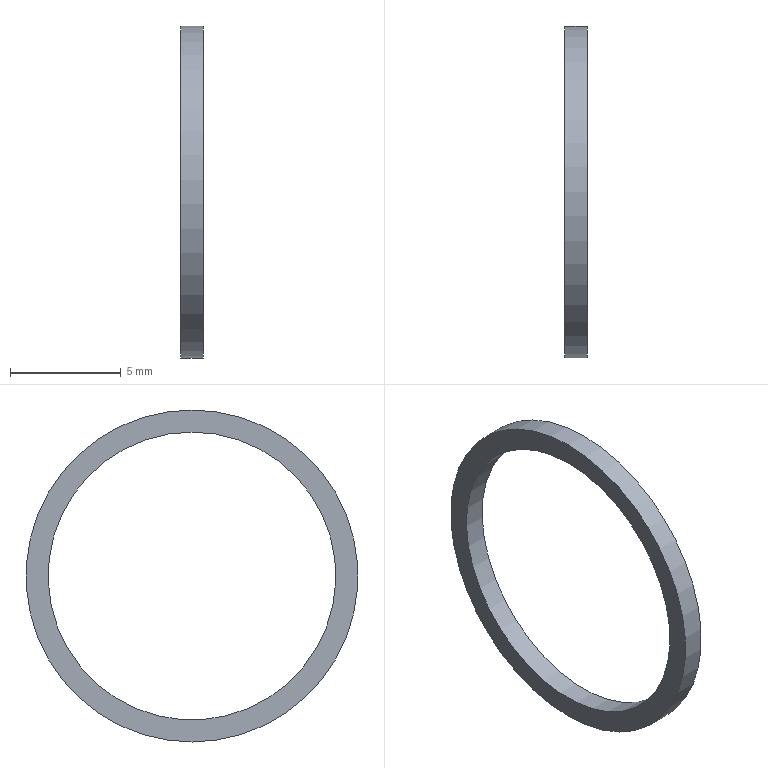Component | NX | WASHER | 1 solid | 4 faces | box 1 x 15 x 15 mm | volume 44 mm3 | plane 2 | cylinder 2 | commonest cylinder face diameters 15 x1 13 x1
STEP:
#1=CARTESIAN_POINT('',(0.,0.,0.));
#2=DIRECTION('',(0.,0.,1.));
#3=DIRECTION('',(1.,0.,0.));
#4=AXIS2_PLACEMENT_3D('',#1,#2,#3);
#5=CARTESIAN_POINT('',(-14.772,-17.527,-182.219));
#6=VERTEX_POINT('',#5);
#7=CARTESIAN_POINT('',(-14.772,-17.527,-188.719));
#8=DIRECTION('',(-1.,0.,0.));
#9=DIRECTION('',(0.,0.,1.));
#10=AXIS2_PLACEMENT_3D('',#7,#8,#9);
#11=CIRCLE('',#10,6.5);
#12=CARTESIAN_POINT('',(-14.772,-17.527,-188.719));
#13=DIRECTION('',(1.,0.,0.));
#14=DIRECTION('',(0.,0.,-1.));
#15=AXIS2_PLACEMENT_3D('',#12,#13,#14);
#16=PLANE('',#15);
#17=CARTESIAN_POINT('',(-6.5,0.));
#18=CARTESIAN_POINT('',(-6.5,11.258));
#19=CARTESIAN_POINT('',(3.25,5.629));
#20=CARTESIAN_POINT('',(13.,0.));
#21=CARTESIAN_POINT('',(3.25,-5.629));
#22=CARTESIAN_POINT('',(-6.5,-11.258));
#23=CARTESIAN_POINT('',(-6.5,0.));
#24=(BOUNDED_CURVE()B_SPLINE_CURVE(2,(#17,#18,#19,#20,#21,#22,#23),.UNSPECIFIED.,.T.,.F.)B_SPLINE_CURVE_WITH_KNOTS((1,2,2,2,2,1),(-2.094,0.,2.094,4.189,6.283,8.378),.UNSPECIFIED.)CURVE()GEOMETRIC_REPRESENTATION_ITEM()RATIONAL_B_SPLINE_CURVE((1.,0.5,1.,0.5,1.,0.5,1.))REPRESENTATION_ITEM(''));
#25=(GEOMETRIC_REPRESENTATION_CONTEXT(2)PARAMETRIC_REPRESENTATION_CONTEXT()REPRESENTATION_CONTEXT('',''));
#26=DEFINITIONAL_REPRESENTATION('',(#24),#25);
#27=PCURVE('',#16,#26);
#28=CARTESIAN_POINT('',(-14.772,-17.527,-188.719));
#29=DIRECTION('',(-1.,0.,0.));
#30=DIRECTION('',(0.,0.,1.));
#31=AXIS2_PLACEMENT_3D('',#28,#29,#30);
#32=CYLINDRICAL_SURFACE('',#31,6.5);
#33=CARTESIAN_POINT('',(0.,0.));
#34=DIRECTION('',(1.,0.));
#35=VECTOR('',#34,1.);
#36=LINE('',#33,#35);
#37=(GEOMETRIC_REPRESENTATION_CONTEXT(2)PARAMETRIC_REPRESENTATION_CONTEXT()REPRESENTATION_CONTEXT('',''));
#38=DEFINITIONAL_REPRESENTATION('',(#36),#37);
#39=PCURVE('',#32,#38);
#40=SURFACE_CURVE('',#11,(#27,#39),.PCURVE_S1.);
#41=EDGE_CURVE('',#6,#6,#40,.T.);
#42=ORIENTED_EDGE('',*,*,#41,.T.);
#43=EDGE_LOOP('',(#42));
#44=FACE_BOUND('',#43,.T.);
#45=CARTESIAN_POINT('',(-14.772,-17.527,-196.219));
#46=VERTEX_POINT('',#45);
#47=CARTESIAN_POINT('',(-14.772,-17.527,-188.719));
#48=DIRECTION('',(-1.,0.,0.));
#49=DIRECTION('',(0.,0.,-1.));
#50=AXIS2_PLACEMENT_3D('',#47,#48,#49);
#51=CIRCLE('',#50,7.5);
#52=CARTESIAN_POINT('',(7.5,0.));
#53=CARTESIAN_POINT('',(7.5,-12.99));
#54=CARTESIAN_POINT('',(-3.75,-6.495));
#55=CARTESIAN_POINT('',(-15.,-0.));
#56=CARTESIAN_POINT('',(-3.75,6.495));
#57=CARTESIAN_POINT('',(7.5,12.99));
#58=CARTESIAN_POINT('',(7.5,0.));
#59=(BOUNDED_CURVE()B_SPLINE_CURVE(2,(#52,#53,#54,#55,#56,#57,#58),.UNSPECIFIED.,.T.,.F.)B_SPLINE_CURVE_WITH_KNOTS((1,2,2,2,2,1),(-2.094,0.,2.094,4.189,6.283,8.378),.UNSPECIFIED.)CURVE()GEOMETRIC_REPRESENTATION_ITEM()RATIONAL_B_SPLINE_CURVE((1.,0.5,1.,0.5,1.,0.5,1.))REPRESENTATION_ITEM(''));
#60=(GEOMETRIC_REPRESENTATION_CONTEXT(2)PARAMETRIC_REPRESENTATION_CONTEXT()REPRESENTATION_CONTEXT('',''));
#61=DEFINITIONAL_REPRESENTATION('',(#59),#60);
#62=PCURVE('',#16,#61);
#63=CARTESIAN_POINT('',(-15.772,-17.527,-188.719));
#64=DIRECTION('',(1.,0.,0.));
#65=DIRECTION('',(0.,0.,-1.));
#66=AXIS2_PLACEMENT_3D('',#63,#64,#65);
#67=CYLINDRICAL_SURFACE('',#66,7.5);
#68=CARTESIAN_POINT('',(6.283,1.));
#69=DIRECTION('',(-1.,0.));
#70=VECTOR('',#69,1.);
#71=LINE('',#68,#70);
#72=(GEOMETRIC_REPRESENTATION_CONTEXT(2)PARAMETRIC_REPRESENTATION_CONTEXT()REPRESENTATION_CONTEXT('',''));
#73=DEFINITIONAL_REPRESENTATION('',(#71),#72);
#74=PCURVE('',#67,#73);
#75=SURFACE_CURVE('',#51,(#62,#74),.PCURVE_S1.);
#76=EDGE_CURVE('',#46,#46,#75,.T.);
#77=ORIENTED_EDGE('',*,*,#76,.F.);
#78=EDGE_LOOP('',(#77));
#79=FACE_BOUND('',#78,.T.);
#80=ADVANCED_FACE('',(#44,#79),#16,.T.);
#81=CARTESIAN_POINT('',(-15.772,-17.527,-182.219));
#82=VERTEX_POINT('',#81);
#83=CARTESIAN_POINT('',(-15.772,-17.527,-188.719));
#84=DIRECTION('',(-1.,0.,0.));
#85=DIRECTION('',(0.,0.,1.));
#86=AXIS2_PLACEMENT_3D('',#83,#84,#85);
#87=CIRCLE('',#86,6.5);
#88=CARTESIAN_POINT('',(-15.772,-17.527,-188.719));
#89=DIRECTION('',(-1.,0.,0.));
#90=DIRECTION('',(0.,0.,1.));
#91=AXIS2_PLACEMENT_3D('',#88,#89,#90);
#92=PLANE('',#91);
#93=CARTESIAN_POINT('',(0.,0.));
#94=DIRECTION('',(1.,0.));
#95=AXIS2_PLACEMENT_2D('',#93,#94);
#96=CIRCLE('',#95,6.5);
#97=(GEOMETRIC_REPRESENTATION_CONTEXT(2)PARAMETRIC_REPRESENTATION_CONTEXT()REPRESENTATION_CONTEXT('',''));
#98=DEFINITIONAL_REPRESENTATION('',(#96),#97);
#99=PCURVE('',#92,#98);
#100=CARTESIAN_POINT('',(0.,1.));
#101=DIRECTION('',(1.,0.));
#102=VECTOR('',#101,1.);
#103=LINE('',#100,#102);
#104=(GEOMETRIC_REPRESENTATION_CONTEXT(2)PARAMETRIC_REPRESENTATION_CONTEXT()REPRESENTATION_CONTEXT('',''));
#105=DEFINITIONAL_REPRESENTATION('',(#103),#104);
#106=PCURVE('',#32,#105);
#107=SURFACE_CURVE('',#87,(#99,#106),.PCURVE_S1.);
#108=EDGE_CURVE('',#82,#82,#107,.T.);
#109=ORIENTED_EDGE('',*,*,#108,.F.);
#110=EDGE_LOOP('',(#109));
#111=FACE_BOUND('',#110,.T.);
#112=CARTESIAN_POINT('',(-15.772,-17.527,-196.219));
#113=VERTEX_POINT('',#112);
#114=CARTESIAN_POINT('',(-15.772,-17.527,-188.719));
#115=DIRECTION('',(1.,0.,0.));
#116=DIRECTION('',(0.,0.,-1.));
#117=AXIS2_PLACEMENT_3D('',#114,#115,#116);
#118=CIRCLE('',#117,7.5);
#119=CARTESIAN_POINT('',(-7.5,0.));
#120=CARTESIAN_POINT('',(-7.5,12.99));
#121=CARTESIAN_POINT('',(3.75,6.495));
#122=CARTESIAN_POINT('',(15.,0.));
#123=CARTESIAN_POINT('',(3.75,-6.495));
#124=CARTESIAN_POINT('',(-7.5,-12.99));
#125=CARTESIAN_POINT('',(-7.5,0.));
#126=(BOUNDED_CURVE()B_SPLINE_CURVE(2,(#119,#120,#121,#122,#123,#124,#125),.UNSPECIFIED.,.T.,.F.)B_SPLINE_CURVE_WITH_KNOTS((1,2,2,2,2,1),(-2.094,0.,2.094,4.189,6.283,8.378),.UNSPECIFIED.)CURVE()GEOMETRIC_REPRESENTATION_ITEM()RATIONAL_B_SPLINE_CURVE((1.,0.5,1.,0.5,1.,0.5,1.))REPRESENTATION_ITEM(''));
#127=(GEOMETRIC_REPRESENTATION_CONTEXT(2)PARAMETRIC_REPRESENTATION_CONTEXT()REPRESENTATION_CONTEXT('',''));
#128=DEFINITIONAL_REPRESENTATION('',(#126),#127);
#129=PCURVE('',#92,#128);
#130=CARTESIAN_POINT('',(0.,0.));
#131=DIRECTION('',(1.,0.));
#132=VECTOR('',#131,1.);
#133=LINE('',#130,#132);
#134=(GEOMETRIC_REPRESENTATION_CONTEXT(2)PARAMETRIC_REPRESENTATION_CONTEXT()REPRESENTATION_CONTEXT('',''));
#135=DEFINITIONAL_REPRESENTATION('',(#133),#134);
#136=PCURVE('',#67,#135);
#137=SURFACE_CURVE('',#118,(#129,#136),.PCURVE_S1.);
#138=EDGE_CURVE('',#113,#113,#137,.T.);
#139=ORIENTED_EDGE('',*,*,#138,.F.);
#140=EDGE_LOOP('',(#139));
#141=FACE_BOUND('',#140,.T.);
#142=ADVANCED_FACE('',(#111,#141),#92,.T.);
#143=ORIENTED_EDGE('',*,*,#76,.T.);
#144=CARTESIAN_POINT('',(-15.772,-17.527,-196.219));
#145=CARTESIAN_POINT('',(-14.772,-17.527,-196.219));
#146=B_SPLINE_CURVE_WITH_KNOTS('',1,(#144,#145),.UNSPECIFIED.,.F.,.F.,(2,2),(0.,1.),.PIECEWISE_BEZIER_KNOTS.);
#147=CARTESIAN_POINT('',(0.,0.));
#148=DIRECTION('',(0.,1.));
#149=VECTOR('',#148,1.);
#150=LINE('',#147,#149);
#151=(GEOMETRIC_REPRESENTATION_CONTEXT(2)PARAMETRIC_REPRESENTATION_CONTEXT()REPRESENTATION_CONTEXT('',''));
#152=DEFINITIONAL_REPRESENTATION('',(#150),#151);
#153=PCURVE('',#67,#152);
#154=CARTESIAN_POINT('',(6.283,0.));
#155=DIRECTION('',(0.,1.));
#156=VECTOR('',#155,1.);
#157=LINE('',#154,#156);
#158=(GEOMETRIC_REPRESENTATION_CONTEXT(2)PARAMETRIC_REPRESENTATION_CONTEXT()REPRESENTATION_CONTEXT('',''));
#159=DEFINITIONAL_REPRESENTATION('',(#157),#158);
#160=PCURVE('',#67,#159);
#161=SEAM_CURVE('',#146,(#153,#160),.PCURVE_S1.);
#162=EDGE_CURVE('',#113,#46,#161,.T.);
#163=ORIENTED_EDGE('',*,*,#162,.F.);
#164=ORIENTED_EDGE('',*,*,#138,.T.);
#165=ORIENTED_EDGE('',*,*,#162,.T.);
#166=EDGE_LOOP('',(#143,#163,#164,#165));
#167=FACE_BOUND('',#166,.T.);
#168=ADVANCED_FACE('',(#167),#67,.T.);
#169=ORIENTED_EDGE('',*,*,#108,.F.);
#170=CARTESIAN_POINT('',(-14.772,-17.527,-182.219));
#171=CARTESIAN_POINT('',(-15.772,-17.527,-182.219));
#172=B_SPLINE_CURVE_WITH_KNOTS('',1,(#170,#171),.UNSPECIFIED.,.F.,.F.,(2,2),(0.,1.),.PIECEWISE_BEZIER_KNOTS.);
#173=CARTESIAN_POINT('',(0.,0.));
#174=DIRECTION('',(0.,1.));
#175=VECTOR('',#174,1.);
#176=LINE('',#173,#175);
#177=(GEOMETRIC_REPRESENTATION_CONTEXT(2)PARAMETRIC_REPRESENTATION_CONTEXT()REPRESENTATION_CONTEXT('',''));
#178=DEFINITIONAL_REPRESENTATION('',(#176),#177);
#179=PCURVE('',#32,#178);
#180=CARTESIAN_POINT('',(6.283,0.));
#181=DIRECTION('',(0.,1.));
#182=VECTOR('',#181,1.);
#183=LINE('',#180,#182);
#184=(GEOMETRIC_REPRESENTATION_CONTEXT(2)PARAMETRIC_REPRESENTATION_CONTEXT()REPRESENTATION_CONTEXT('',''));
#185=DEFINITIONAL_REPRESENTATION('',(#183),#184);
#186=PCURVE('',#32,#185);
#187=SEAM_CURVE('',#172,(#179,#186),.PCURVE_S1.);
#188=EDGE_CURVE('',#6,#82,#187,.T.);
#189=ORIENTED_EDGE('',*,*,#188,.F.);
#190=ORIENTED_EDGE('',*,*,#41,.T.);
#191=ORIENTED_EDGE('',*,*,#188,.T.);
#192=EDGE_LOOP('',(#169,#189,#190,#191));
#193=FACE_BOUND('',#192,.F.);
#194=ADVANCED_FACE('',(#193),#32,.F.);
#195=CLOSED_SHELL('',(#80,#142,#168,#194));
#196=MANIFOLD_SOLID_BREP('',#195);
#197=(LENGTH_UNIT()NAMED_UNIT(*)SI_UNIT(.MILLI.,.METRE.));
#198=UNCERTAINTY_MEASURE_WITH_UNIT(LENGTH_MEASURE(0.00001),#197,'','');
#199=(NAMED_UNIT(*)PLANE_ANGLE_UNIT()SI_UNIT($,.RADIAN.));
#200=(NAMED_UNIT(*)SI_UNIT($,.STERADIAN.)SOLID_ANGLE_UNIT());
#201=(GEOMETRIC_REPRESENTATION_CONTEXT(3)GLOBAL_UNCERTAINTY_ASSIGNED_CONTEXT((#198))GLOBAL_UNIT_ASSIGNED_CONTEXT((#197,#199,#200))REPRESENTATION_CONTEXT('',''));
#202=ADVANCED_BREP_SHAPE_REPRESENTATION('',(#4,#196),#201);